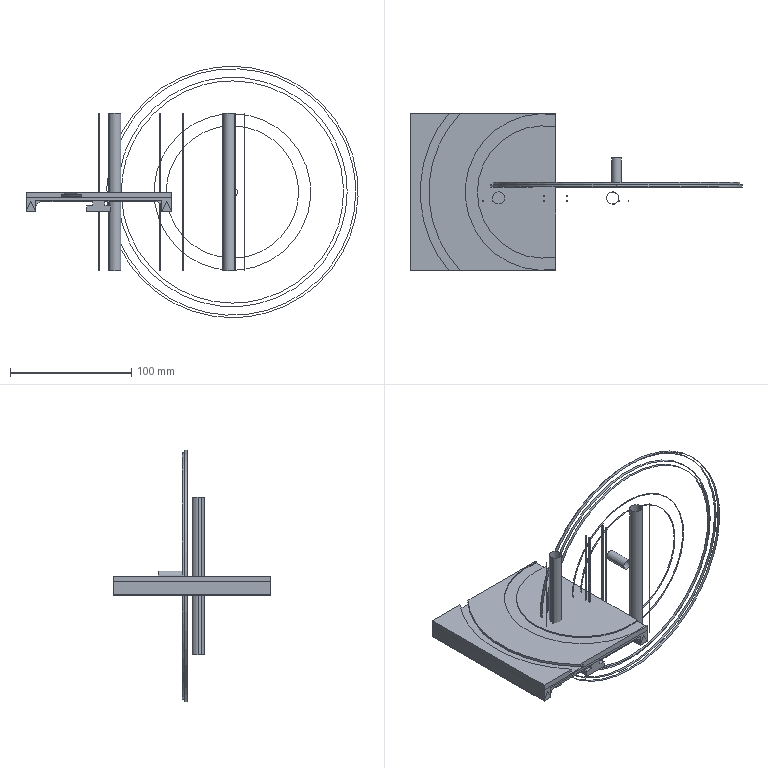CAM job | Mastercam | mm | 13 operations | part box 273.5 x 130 x 207
1. Contour (Ramp) | 4 - 6 平铣刀
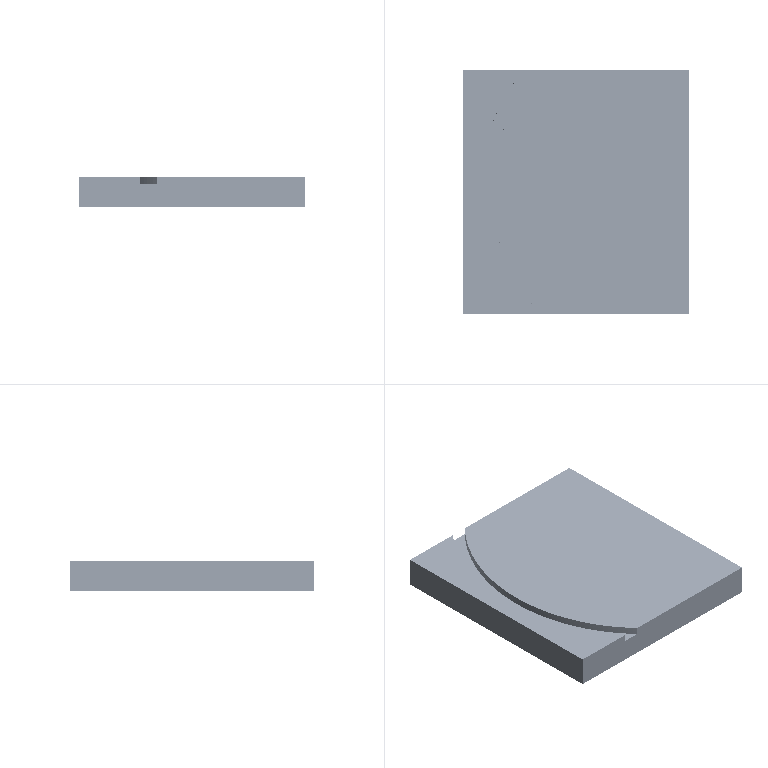2. Contour (Ramp) | 4 - 6 平铣刀
3. Contour (2D) | 5 - 6 平铣刀
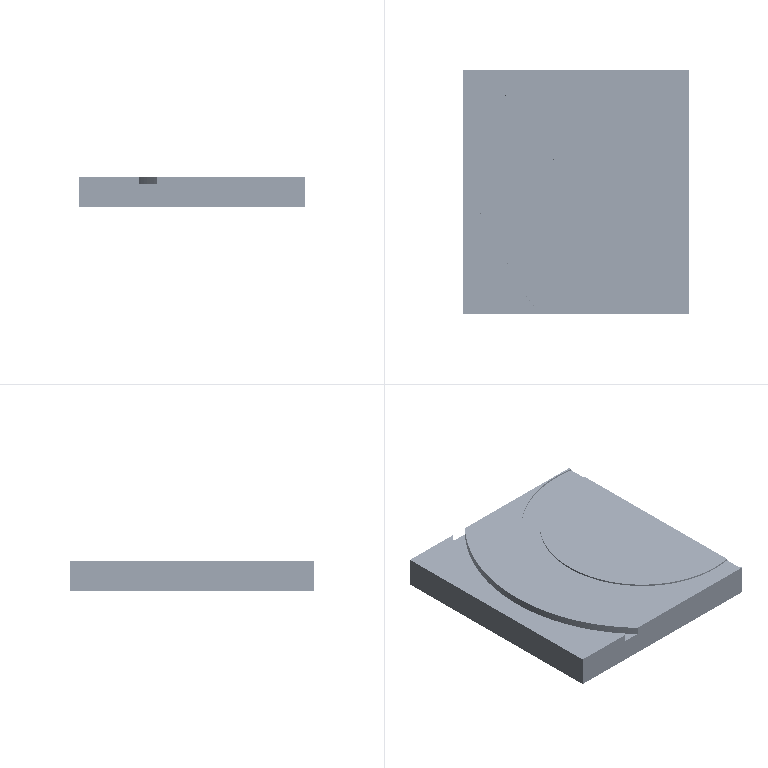4. Contour (2D) | 4 - 6 平铣刀
5. Contour (2D) | 1 - 11 槽铣刀或锯式刀具
6. Model Chamfer | 6 - 6 倒角刀
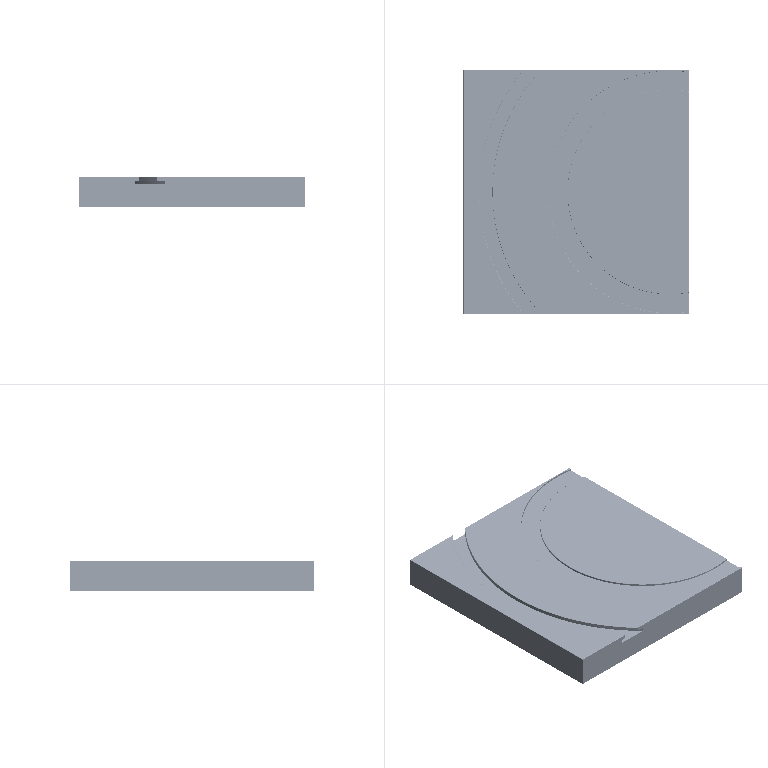7. Surface Rough Pocket | 2 - 12 平铣刀
8. 2D High Speed (2D Area Mill) | 3 - 12 平铣刀
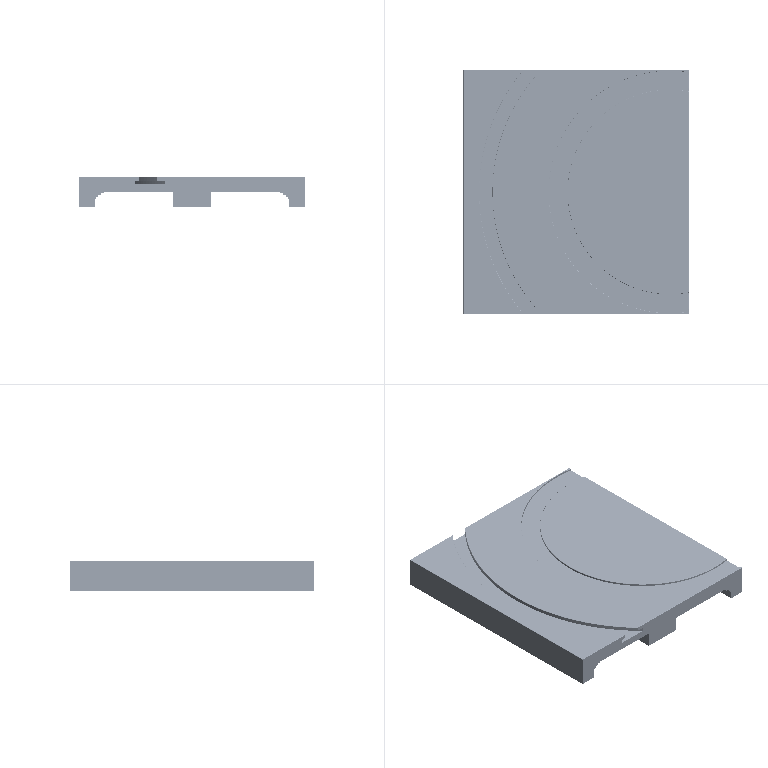9. Contour (2D) | 3 - 12 平铣刀
10. Contour (2D) | 3 - 12 平铣刀
11. Surface Finish Flowline | 7 - 17 圆鼻铣刀
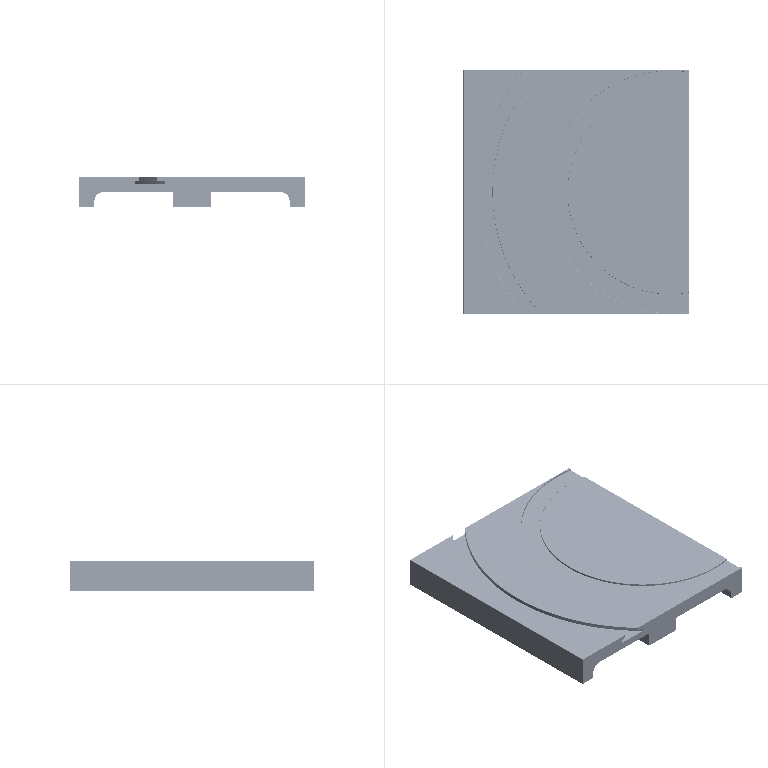12. Surface Finish Flowline | 7 - 17 圆鼻铣刀
13. Contour (2D) | 8 - 20 槽铣刀或锯式刀具